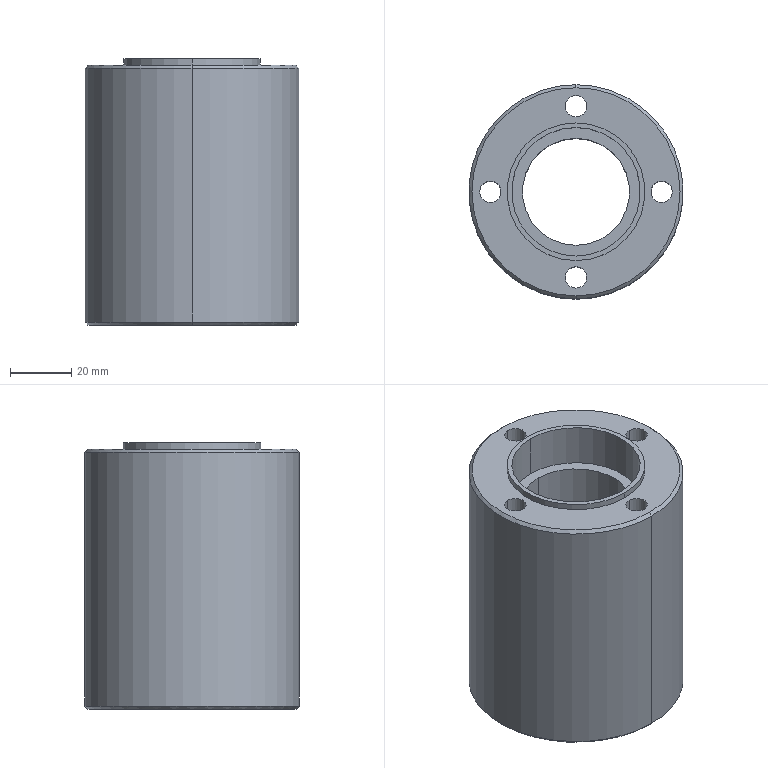Component | SolidWorks | TractionDriveWheelAssembly-1_TractionDriveWheelBearingHousing-2 | 1 solid | 41 faces | box 70 x 70 x 87 mm | volume 214302 mm3 | cylinder 26 | plane 9 | cone 6 | commonest cylinder face diameters 11 x8 7 x8 42 x4 45 x2 70 x2 35 x2
build123d program:
from build123d import *

# Parameters (mm, degrees)
CHAMFER1_SIZE                                       = 1
CHAMFER2_SIZE                                       = 1
CYLINDRICAL_COUNTERSUNK_HOLE_FOR_M6_HEX_D           = 7
CYLINDRICAL_COUNTERSUNK_HOLE_FOR_M6_HEX_CBORE_D     = 11
CYLINDRICAL_COUNTERSUNK_HOLE_FOR_M6_HEX_CBORE_DEPTH = 35
CIRPATTERN1_COUNT                                   = 4
SKETCH5_R                                           = 22.5
SKETCH5_R_2                                         = 21
BOSS_EXTRUDE1_DEPTH                                 = 2


with BuildPart() as part:
    # Sketch1 → Revolve1 (revolve)
    with BuildSketch(Plane.XY, mode=Mode.PRIVATE) as revolve1_sk:
        Polygon((0, 35), (85, 35), (85, 21), (73, 21), (73, 17.5), (12, 17.5), (12, 21), (0, 21), align=None)
    revolve(revolve1_sk.sketch.rotate(Axis((-765.169, 0, 0), (1, 0, 0)), 90), axis=Axis((-765.169, 0, 0), (1, 0, 0)))

    # Chamfer1
    chamfer1_edges = [part.edges().sort_by_distance(p)[0] for p in [
        (0, 0, -21),
    ]]
    chamfer(chamfer1_edges, length=CHAMFER1_SIZE)

    # Chamfer2
    chamfer2_edges = [part.edges().sort_by_distance(p)[0] for p in [
        (0, 0, -35),
        (85, 0, -35),
    ]]
    chamfer(chamfer2_edges, length=CHAMFER2_SIZE)

    # Cylindrical Countersunk Hole for M6 Hex (through all)
    with Locations(Plane.ZY):
        with Locations((0, 28)):
            cylindrical_countersunk_hole_for_m6_hex = CounterBoreHole(CYLINDRICAL_COUNTERSUNK_HOLE_FOR_M6_HEX_D / 2, CYLINDRICAL_COUNTERSUNK_HOLE_FOR_M6_HEX_CBORE_D / 2, CYLINDRICAL_COUNTERSUNK_HOLE_FOR_M6_HEX_CBORE_DEPTH)

    # CirPattern1: Cylindrical Countersunk Hole for M6 Hex ×4 about axis
    cirpattern1_axis = Axis((0, 0, 0), (1, 0, 0))
    for i in range(1, CIRPATTERN1_COUNT):
        add(cylindrical_countersunk_hole_for_m6_hex.rotate(cirpattern1_axis, i * 360 / CIRPATTERN1_COUNT), mode=Mode.SUBTRACT)

    # Sketch5 → Boss-Extrude1 (add)
    with BuildSketch(Plane(origin=(85, 0, 0), x_dir=(0, 0, -1), z_dir=(1, 0, 0))):
        with Locations(Location((0, 0, 0), (0, 0, 180))):
            Circle(SKETCH5_R)
        with Locations(Location((0, 0, 0), (0, 0, 180))):
            Circle(SKETCH5_R_2, mode=Mode.SUBTRACT)
    extrude(amount=BOSS_EXTRUDE1_DEPTH)


solid = part.part

# Placed as in the assembly
solid = solid.moved(Location((-299.507, -39.911, 410), (0, -90, 0)))